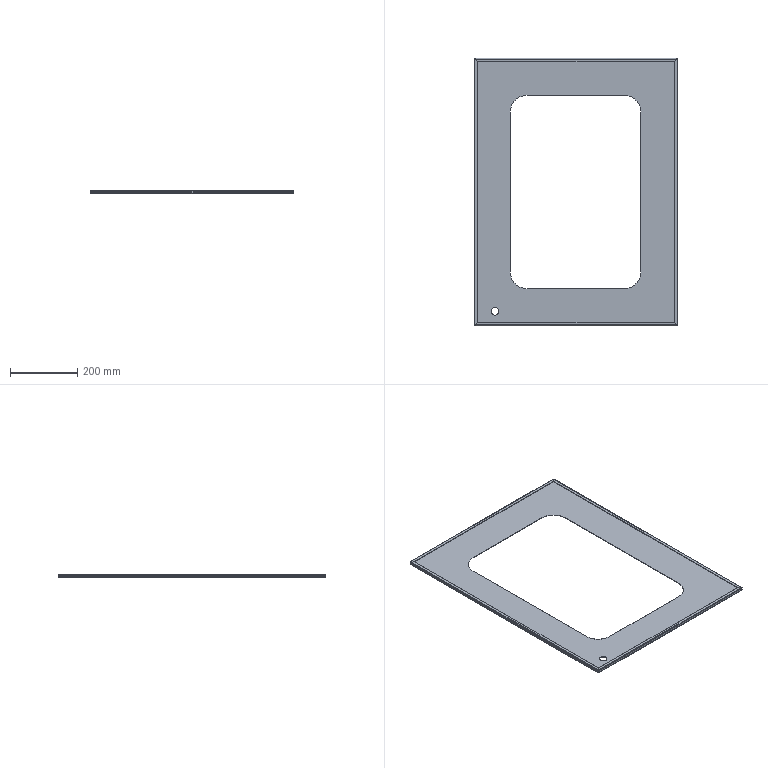Component | SolidWorks | UpperDoorFrame-1_ElectricalControlMountingPlate-1 | 1 solid | 80 faces | volume 456517 mm3 | plane 42 | cylinder 22 | spline 16 | commonest cylinder face diameters 4.473 x8 1.473 x8 100 x4 22 x2